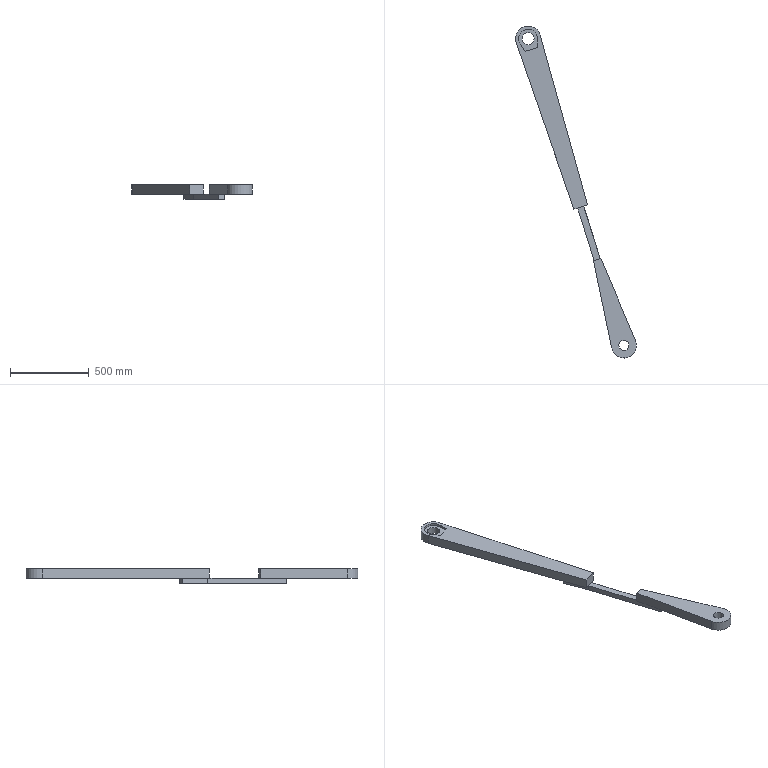Component | NX | TIE_ROD | 1 solid | 26 faces | volume 13544065 mm3 | plane 21 | cylinder 5 | commonest cylinder face diameters 160 x2 76 x1 64 x1 120 x1